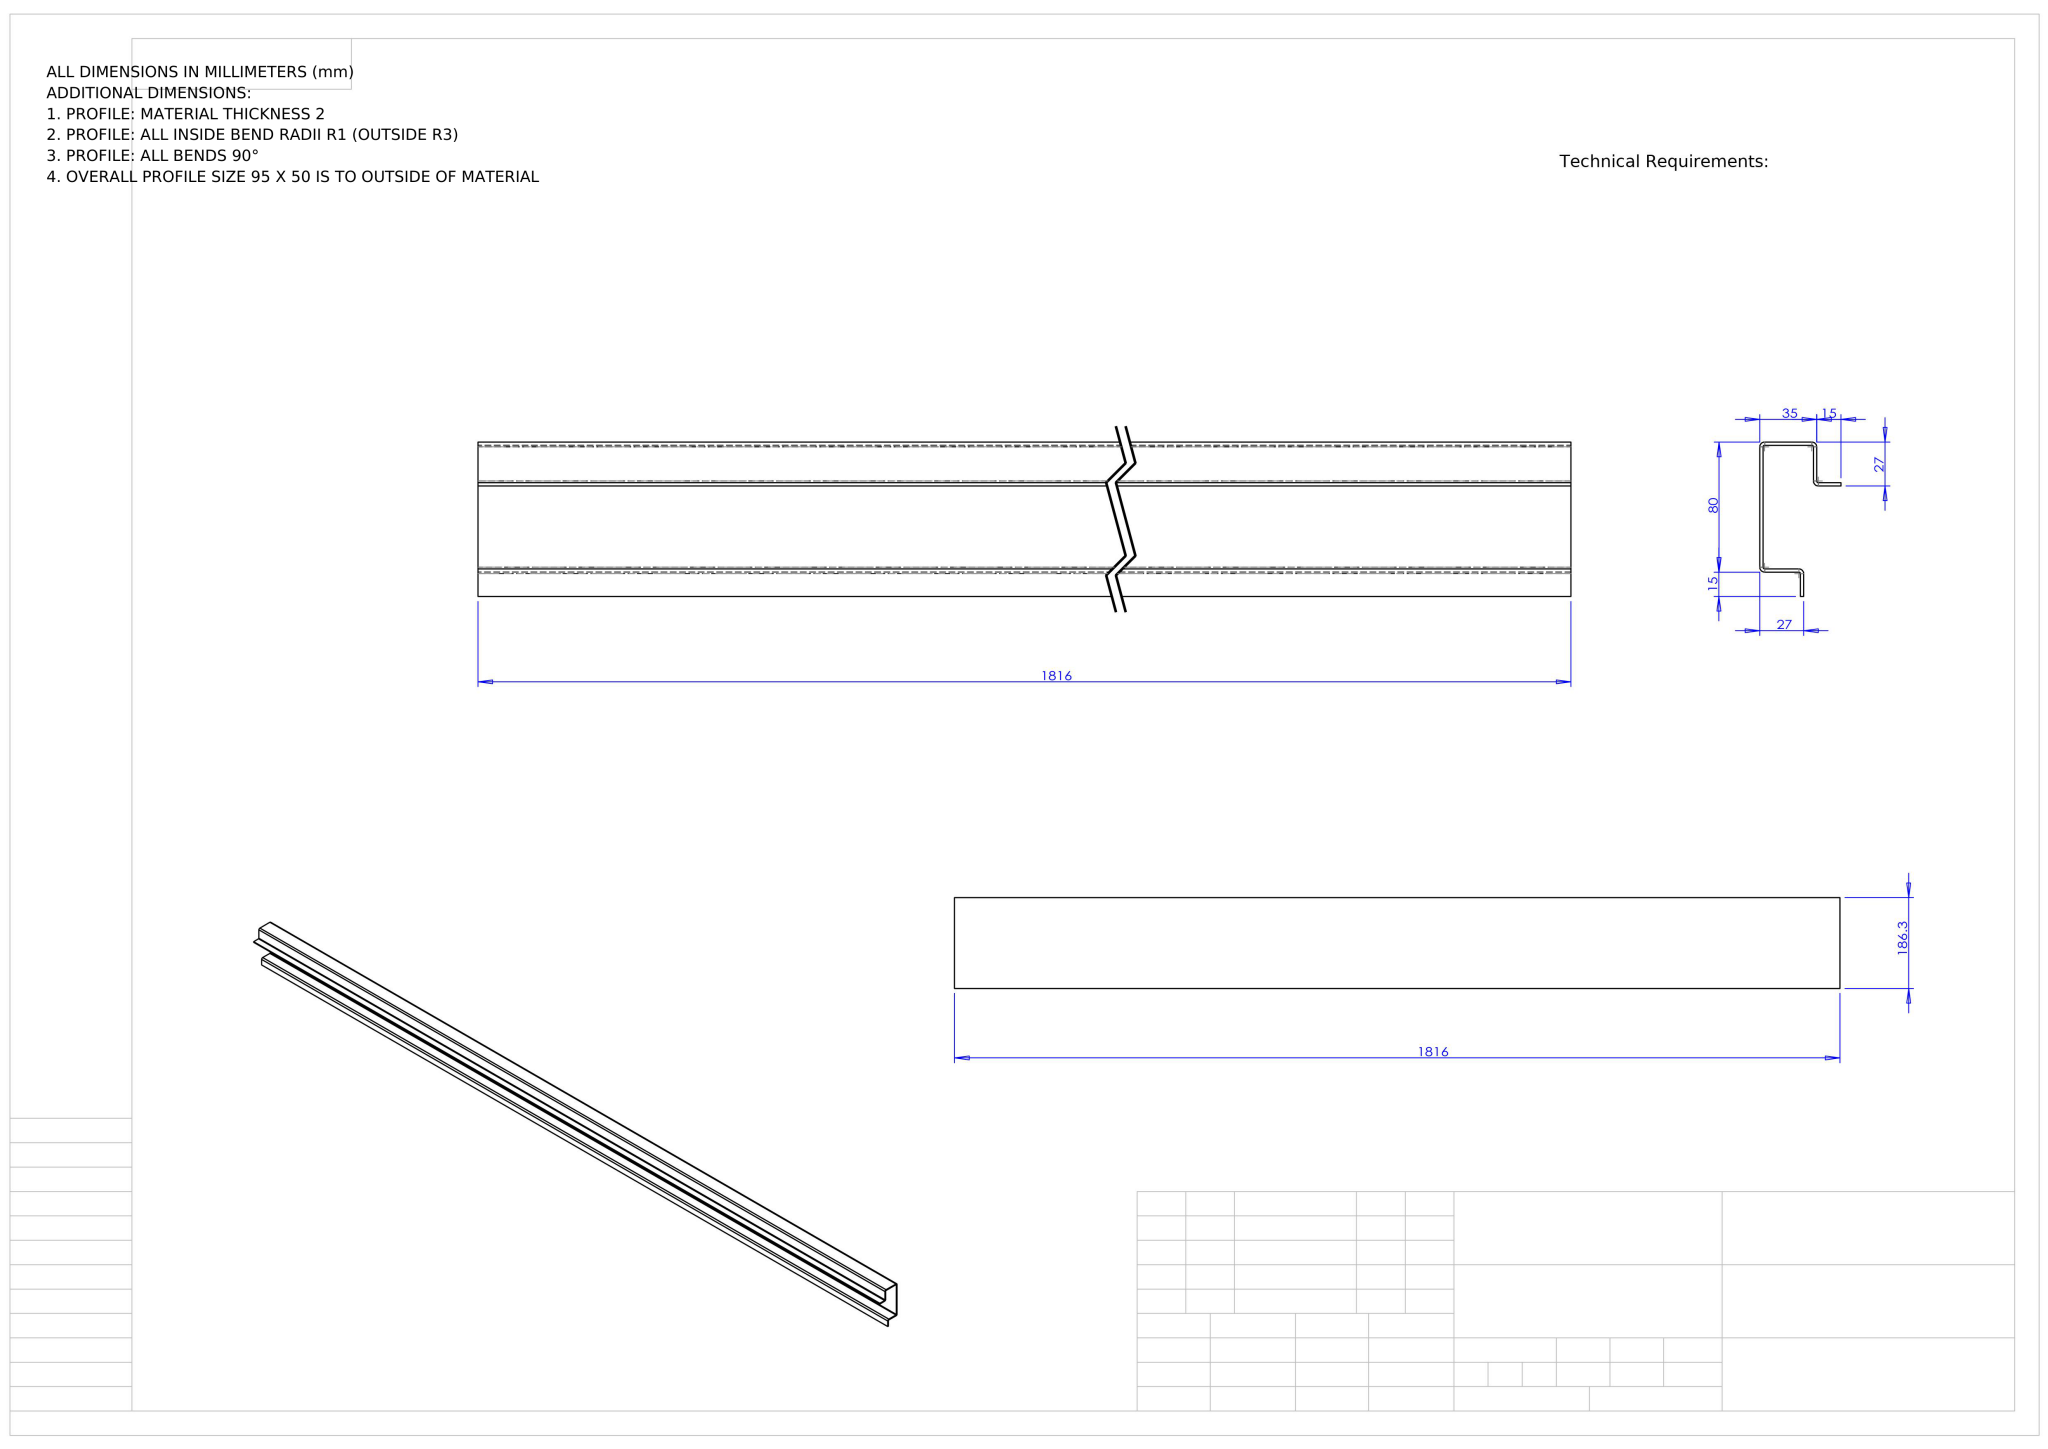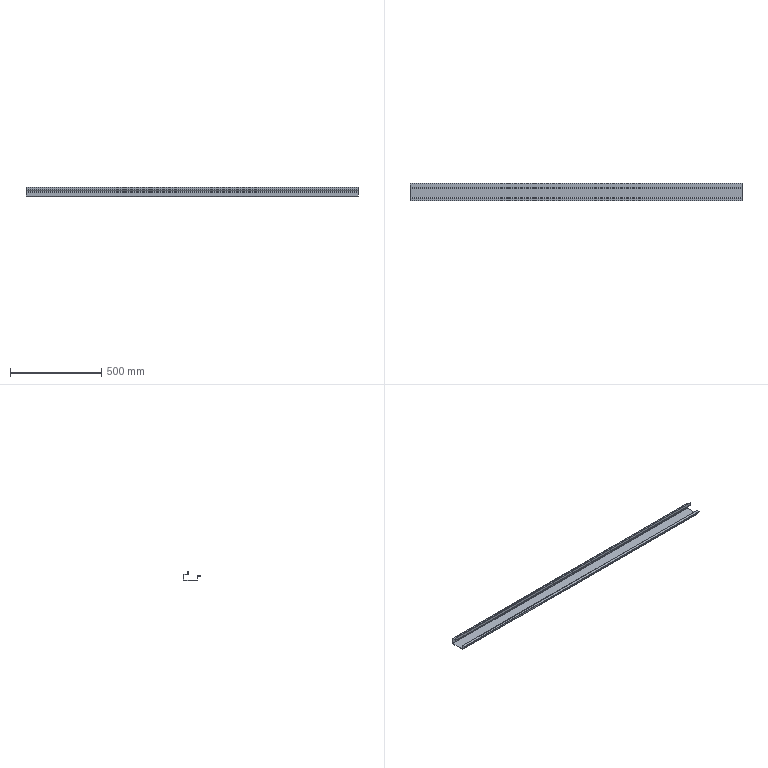Part | NX | mm | 1 solid | 46 faces | box 1816 x 95 x 50 mm | volume 685387 mm3 | plane 36 | cylinder 10 | commonest cylinder face diameters 2 x5 6 x5